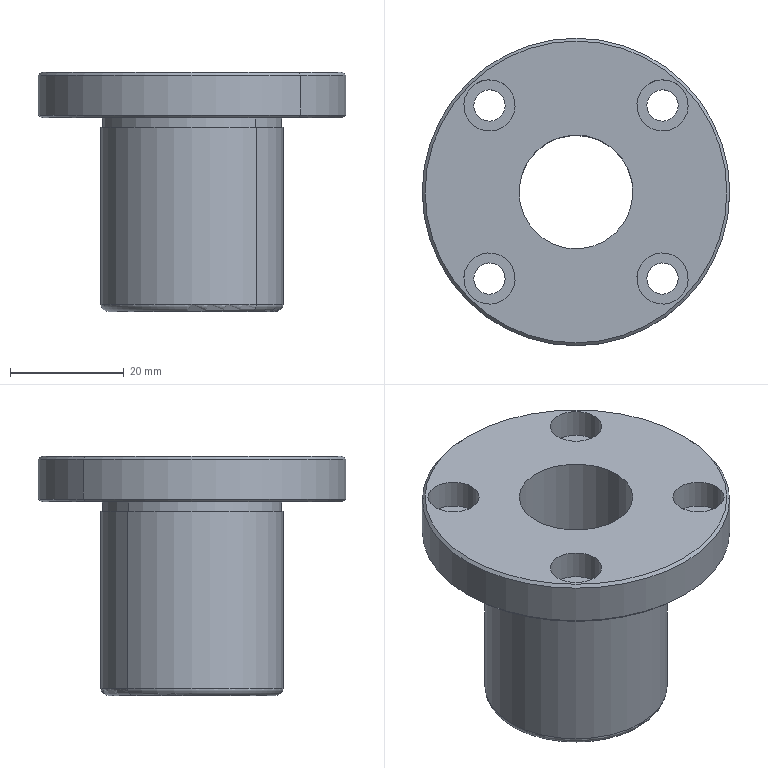Component | SolidWorks | SL010-RightStreamline-1-1_SL010-C-LHFR20-2-1-1 | 1 solid | 38 faces | box 54 x 54 x 42 mm | volume 30780 mm3 | cylinder 24 | plane 8 | cone 4 | torus 2 | commonest cylinder face diameters 9 x8 5.5 x8 54 x2 31.5 x2 32 x2 20 x2
STEP:
#1=COLOUR_RGB('',0.7922,0.8196,0.9333);
#2=FILL_AREA_STYLE_COLOUR('',#1);
#3=FILL_AREA_STYLE('',(#2));
#4=SURFACE_STYLE_FILL_AREA(#3);
#5=SURFACE_SIDE_STYLE('',(#4));
#6=SURFACE_STYLE_USAGE(.BOTH.,#5);
#7=PRESENTATION_STYLE_ASSIGNMENT((#6));
#8=CARTESIAN_POINT('',(27.442,-8.344,-12.328));
#9=VERTEX_POINT('',#8);
#10=CARTESIAN_POINT('',(27.692,-8.594,-12.328));
#11=VERTEX_POINT('',#10);
#12=CARTESIAN_POINT('',(27.567,-8.469,-12.328));
#13=DIRECTION('',(0.,0.,1.));
#14=DIRECTION('',(0.7071,-0.7071,0.));
#15=AXIS2_PLACEMENT_3D('',#12,#13,#14);
#16=CIRCLE('',#15,0.1772);
#17=EDGE_CURVE('',#9,#11,#16,.T.);
#18=ORIENTED_EDGE('',*,*,#17,.F.);
#19=CARTESIAN_POINT('',(27.442,-8.344,-12.127));
#20=VERTEX_POINT('',#19);
#21=CARTESIAN_POINT('',(27.442,-8.344,-12.127));
#22=DIRECTION('',(0.,0.,1.));
#23=VECTOR('',#22,39.37);
#24=LINE('',#21,#23);
#25=EDGE_CURVE('',#9,#20,#24,.T.);
#26=ORIENTED_EDGE('',*,*,#25,.T.);
#27=CARTESIAN_POINT('',(27.692,-8.594,-12.127));
#28=VERTEX_POINT('',#27);
#29=CARTESIAN_POINT('',(27.567,-8.469,-12.127));
#30=DIRECTION('',(0.,0.,1.));
#31=DIRECTION('',(0.7071,-0.7071,0.));
#32=AXIS2_PLACEMENT_3D('',#29,#30,#31);
#33=CIRCLE('',#32,0.1772);
#34=EDGE_CURVE('',#20,#28,#33,.T.);
#35=ORIENTED_EDGE('',*,*,#34,.T.);
#36=CARTESIAN_POINT('',(27.692,-8.594,-12.127));
#37=DIRECTION('',(0.,0.,1.));
#38=VECTOR('',#37,39.37);
#39=LINE('',#36,#38);
#40=EDGE_CURVE('',#11,#28,#39,.T.);
#41=ORIENTED_EDGE('',*,*,#40,.F.);
#42=EDGE_LOOP('',(#18,#26,#35,#41));
#43=FACE_OUTER_BOUND('',#42,.T.);
#44=CARTESIAN_POINT('',(27.567,-8.469,-12.127));
#45=DIRECTION('',(0.,0.,1.));
#46=DIRECTION('',(0.7071,-0.7071,0.));
#47=AXIS2_PLACEMENT_3D('',#44,#45,#46);
#48=CYLINDRICAL_SURFACE('',#47,0.1772);
#49=ADVANCED_FACE('',(#43),#48,.F.);
#50=CARTESIAN_POINT('',(27.49,-8.392,-12.442));
#51=VERTEX_POINT('',#50);
#52=CARTESIAN_POINT('',(27.644,-8.545,-12.442));
#53=VERTEX_POINT('',#52);
#54=CARTESIAN_POINT('',(27.567,-8.469,-12.442));
#55=DIRECTION('',(0.,0.,1.));
#56=DIRECTION('',(0.7071,-0.7071,0.));
#57=AXIS2_PLACEMENT_3D('',#54,#55,#56);
#58=CIRCLE('',#57,0.1083);
#59=EDGE_CURVE('',#51,#53,#58,.T.);
#60=ORIENTED_EDGE('',*,*,#59,.F.);
#61=CARTESIAN_POINT('',(27.49,-8.392,-12.328));
#62=VERTEX_POINT('',#61);
#63=CARTESIAN_POINT('',(27.49,-8.392,-12.127));
#64=DIRECTION('',(0.,0.,1.));
#65=VECTOR('',#64,39.37);
#66=LINE('',#63,#65);
#67=EDGE_CURVE('',#51,#62,#66,.T.);
#68=ORIENTED_EDGE('',*,*,#67,.T.);
#69=CARTESIAN_POINT('',(27.644,-8.545,-12.328));
#70=VERTEX_POINT('',#69);
#71=CARTESIAN_POINT('',(27.567,-8.469,-12.328));
#72=DIRECTION('',(0.,0.,1.));
#73=DIRECTION('',(0.7071,-0.7071,0.));
#74=AXIS2_PLACEMENT_3D('',#71,#72,#73);
#75=CIRCLE('',#74,0.1083);
#76=EDGE_CURVE('',#62,#70,#75,.T.);
#77=ORIENTED_EDGE('',*,*,#76,.T.);
#78=CARTESIAN_POINT('',(27.644,-8.545,-12.127));
#79=DIRECTION('',(0.,0.,1.));
#80=VECTOR('',#79,39.37);
#81=LINE('',#78,#80);
#82=EDGE_CURVE('',#53,#70,#81,.T.);
#83=ORIENTED_EDGE('',*,*,#82,.F.);
#84=EDGE_LOOP('',(#60,#68,#77,#83));
#85=FACE_OUTER_BOUND('',#84,.T.);
#86=CARTESIAN_POINT('',(27.567,-8.469,-12.127));
#87=DIRECTION('',(0.,0.,1.));
#88=DIRECTION('',(0.7071,-0.7071,0.));
#89=AXIS2_PLACEMENT_3D('',#86,#87,#88);
#90=CYLINDRICAL_SURFACE('',#89,0.1083);
#91=ADVANCED_FACE('',(#85),#90,.F.);
#92=CARTESIAN_POINT('',(26.245,-7.146,-12.328));
#93=VERTEX_POINT('',#92);
#94=CARTESIAN_POINT('',(26.495,-7.397,-12.328));
#95=VERTEX_POINT('',#94);
#96=CARTESIAN_POINT('',(26.37,-7.272,-12.328));
#97=DIRECTION('',(0.,0.,1.));
#98=DIRECTION('',(0.7071,-0.7071,0.));
#99=AXIS2_PLACEMENT_3D('',#96,#97,#98);
#100=CIRCLE('',#99,0.1772);
#101=EDGE_CURVE('',#93,#95,#100,.T.);
#102=ORIENTED_EDGE('',*,*,#101,.F.);
#103=CARTESIAN_POINT('',(26.245,-7.146,-12.127));
#104=VERTEX_POINT('',#103);
#105=CARTESIAN_POINT('',(26.245,-7.146,-12.127));
#106=DIRECTION('',(0.,0.,1.));
#107=VECTOR('',#106,39.37);
#108=LINE('',#105,#107);
#109=EDGE_CURVE('',#93,#104,#108,.T.);
#110=ORIENTED_EDGE('',*,*,#109,.T.);
#111=CARTESIAN_POINT('',(26.495,-7.397,-12.127));
#112=VERTEX_POINT('',#111);
#113=CARTESIAN_POINT('',(26.37,-7.272,-12.127));
#114=DIRECTION('',(0.,0.,1.));
#115=DIRECTION('',(0.7071,-0.7071,0.));
#116=AXIS2_PLACEMENT_3D('',#113,#114,#115);
#117=CIRCLE('',#116,0.1772);
#118=EDGE_CURVE('',#104,#112,#117,.T.);
#119=ORIENTED_EDGE('',*,*,#118,.T.);
#120=CARTESIAN_POINT('',(26.495,-7.397,-12.127));
#121=DIRECTION('',(0.,0.,1.));
#122=VECTOR('',#121,39.37);
#123=LINE('',#120,#122);
#124=EDGE_CURVE('',#95,#112,#123,.T.);
#125=ORIENTED_EDGE('',*,*,#124,.F.);
#126=EDGE_LOOP('',(#102,#110,#119,#125));
#127=FACE_OUTER_BOUND('',#126,.T.);
#128=CARTESIAN_POINT('',(26.37,-7.272,-12.127));
#129=DIRECTION('',(0.,0.,1.));
#130=DIRECTION('',(0.7071,-0.7071,0.));
#131=AXIS2_PLACEMENT_3D('',#128,#129,#130);
#132=CYLINDRICAL_SURFACE('',#131,0.1772);
#133=ADVANCED_FACE('',(#127),#132,.F.);
#134=CARTESIAN_POINT('',(26.293,-7.195,-12.442));
#135=VERTEX_POINT('',#134);
#136=CARTESIAN_POINT('',(26.447,-7.348,-12.442));
#137=VERTEX_POINT('',#136);
#138=CARTESIAN_POINT('',(26.37,-7.272,-12.442));
#139=DIRECTION('',(0.,0.,1.));
#140=DIRECTION('',(0.7071,-0.7071,0.));
#141=AXIS2_PLACEMENT_3D('',#138,#139,#140);
#142=CIRCLE('',#141,0.1083);
#143=EDGE_CURVE('',#135,#137,#142,.T.);
#144=ORIENTED_EDGE('',*,*,#143,.F.);
#145=CARTESIAN_POINT('',(26.293,-7.195,-12.328));
#146=VERTEX_POINT('',#145);
#147=CARTESIAN_POINT('',(26.293,-7.195,-12.127));
#148=DIRECTION('',(0.,0.,1.));
#149=VECTOR('',#148,39.37);
#150=LINE('',#147,#149);
#151=EDGE_CURVE('',#135,#146,#150,.T.);
#152=ORIENTED_EDGE('',*,*,#151,.T.);
#153=CARTESIAN_POINT('',(26.447,-7.348,-12.328));
#154=VERTEX_POINT('',#153);
#155=CARTESIAN_POINT('',(26.37,-7.272,-12.328));
#156=DIRECTION('',(0.,0.,1.));
#157=DIRECTION('',(0.7071,-0.7071,0.));
#158=AXIS2_PLACEMENT_3D('',#155,#156,#157);
#159=CIRCLE('',#158,0.1083);
#160=EDGE_CURVE('',#146,#154,#159,.T.);
#161=ORIENTED_EDGE('',*,*,#160,.T.);
#162=CARTESIAN_POINT('',(26.447,-7.348,-12.127));
#163=DIRECTION('',(0.,0.,1.));
#164=VECTOR('',#163,39.37);
#165=LINE('',#162,#164);
#166=EDGE_CURVE('',#137,#154,#165,.T.);
#167=ORIENTED_EDGE('',*,*,#166,.F.);
#168=EDGE_LOOP('',(#144,#152,#161,#167));
#169=FACE_OUTER_BOUND('',#168,.T.);
#170=CARTESIAN_POINT('',(26.37,-7.272,-12.127));
#171=DIRECTION('',(0.,0.,1.));
#172=DIRECTION('',(0.7071,-0.7071,0.));
#173=AXIS2_PLACEMENT_3D('',#170,#171,#172);
#174=CYLINDRICAL_SURFACE('',#173,0.1083);
#175=ADVANCED_FACE('',(#169),#174,.F.);
#176=CARTESIAN_POINT('',(26.245,-8.344,-12.328));
#177=VERTEX_POINT('',#176);
#178=CARTESIAN_POINT('',(26.495,-8.594,-12.328));
#179=VERTEX_POINT('',#178);
#180=CARTESIAN_POINT('',(26.37,-8.469,-12.328));
#181=DIRECTION('',(0.,0.,1.));
#182=DIRECTION('',(0.7071,-0.7071,0.));
#183=AXIS2_PLACEMENT_3D('',#180,#181,#182);
#184=CIRCLE('',#183,0.1772);
#185=EDGE_CURVE('',#177,#179,#184,.T.);
#186=ORIENTED_EDGE('',*,*,#185,.F.);
#187=CARTESIAN_POINT('',(26.245,-8.344,-12.127));
#188=VERTEX_POINT('',#187);
#189=CARTESIAN_POINT('',(26.245,-8.344,-12.127));
#190=DIRECTION('',(0.,0.,1.));
#191=VECTOR('',#190,39.37);
#192=LINE('',#189,#191);
#193=EDGE_CURVE('',#177,#188,#192,.T.);
#194=ORIENTED_EDGE('',*,*,#193,.T.);
#195=CARTESIAN_POINT('',(26.495,-8.594,-12.127));
#196=VERTEX_POINT('',#195);
#197=CARTESIAN_POINT('',(26.37,-8.469,-12.127));
#198=DIRECTION('',(0.,0.,1.));
#199=DIRECTION('',(0.7071,-0.7071,0.));
#200=AXIS2_PLACEMENT_3D('',#197,#198,#199);
#201=CIRCLE('',#200,0.1772);
#202=EDGE_CURVE('',#188,#196,#201,.T.);
#203=ORIENTED_EDGE('',*,*,#202,.T.);
#204=CARTESIAN_POINT('',(26.495,-8.594,-12.127));
#205=DIRECTION('',(0.,0.,1.));
#206=VECTOR('',#205,39.37);
#207=LINE('',#204,#206);
#208=EDGE_CURVE('',#179,#196,#207,.T.);
#209=ORIENTED_EDGE('',*,*,#208,.F.);
#210=EDGE_LOOP('',(#186,#194,#203,#209));
#211=FACE_OUTER_BOUND('',#210,.T.);
#212=CARTESIAN_POINT('',(26.37,-8.469,-12.127));
#213=DIRECTION('',(0.,0.,1.));
#214=DIRECTION('',(0.7071,-0.7071,0.));
#215=AXIS2_PLACEMENT_3D('',#212,#213,#214);
#216=CYLINDRICAL_SURFACE('',#215,0.1772);
#217=ADVANCED_FACE('',(#211),#216,.F.);
#218=CARTESIAN_POINT('',(26.293,-8.392,-12.442));
#219=VERTEX_POINT('',#218);
#220=CARTESIAN_POINT('',(26.447,-8.545,-12.442));
#221=VERTEX_POINT('',#220);
#222=CARTESIAN_POINT('',(26.37,-8.469,-12.442));
#223=DIRECTION('',(0.,0.,1.));
#224=DIRECTION('',(0.7071,-0.7071,0.));
#225=AXIS2_PLACEMENT_3D('',#222,#223,#224);
#226=CIRCLE('',#225,0.1083);
#227=EDGE_CURVE('',#219,#221,#226,.T.);
#228=ORIENTED_EDGE('',*,*,#227,.F.);
#229=CARTESIAN_POINT('',(26.293,-8.392,-12.328));
#230=VERTEX_POINT('',#229);
#231=CARTESIAN_POINT('',(26.293,-8.392,-12.127));
#232=DIRECTION('',(0.,0.,1.));
#233=VECTOR('',#232,39.37);
#234=LINE('',#231,#233);
#235=EDGE_CURVE('',#219,#230,#234,.T.);
#236=ORIENTED_EDGE('',*,*,#235,.T.);
#237=CARTESIAN_POINT('',(26.447,-8.545,-12.328));
#238=VERTEX_POINT('',#237);
#239=CARTESIAN_POINT('',(26.37,-8.469,-12.328));
#240=DIRECTION('',(0.,0.,1.));
#241=DIRECTION('',(0.7071,-0.7071,0.));
#242=AXIS2_PLACEMENT_3D('',#239,#240,#241);
#243=CIRCLE('',#242,0.1083);
#244=EDGE_CURVE('',#230,#238,#243,.T.);
#245=ORIENTED_EDGE('',*,*,#244,.T.);
#246=CARTESIAN_POINT('',(26.447,-8.545,-12.127));
#247=DIRECTION('',(0.,0.,1.));
#248=VECTOR('',#247,39.37);
#249=LINE('',#246,#248);
#250=EDGE_CURVE('',#221,#238,#249,.T.);
#251=ORIENTED_EDGE('',*,*,#250,.F.);
#252=EDGE_LOOP('',(#228,#236,#245,#251));
#253=FACE_OUTER_BOUND('',#252,.T.);
#254=CARTESIAN_POINT('',(26.37,-8.469,-12.127));
#255=DIRECTION('',(0.,0.,1.));
#256=DIRECTION('',(0.7071,-0.7071,0.));
#257=AXIS2_PLACEMENT_3D('',#254,#255,#256);
#258=CYLINDRICAL_SURFACE('',#257,0.1083);
#259=ADVANCED_FACE('',(#253),#258,.F.);
#260=CARTESIAN_POINT('',(27.442,-7.146,-12.328));
#261=VERTEX_POINT('',#260);
#262=CARTESIAN_POINT('',(27.692,-7.397,-12.328));
#263=VERTEX_POINT('',#262);
#264=CARTESIAN_POINT('',(27.567,-7.272,-12.328));
#265=DIRECTION('',(0.,0.,1.));
#266=DIRECTION('',(0.7071,-0.7071,0.));
#267=AXIS2_PLACEMENT_3D('',#264,#265,#266);
#268=CIRCLE('',#267,0.1772);
#269=EDGE_CURVE('',#261,#263,#268,.T.);
#270=ORIENTED_EDGE('',*,*,#269,.F.);
#271=CARTESIAN_POINT('',(27.442,-7.146,-12.127));
#272=VERTEX_POINT('',#271);
#273=CARTESIAN_POINT('',(27.442,-7.146,-12.127));
#274=DIRECTION('',(0.,0.,1.));
#275=VECTOR('',#274,39.37);
#276=LINE('',#273,#275);
#277=EDGE_CURVE('',#261,#272,#276,.T.);
#278=ORIENTED_EDGE('',*,*,#277,.T.);
#279=CARTESIAN_POINT('',(27.692,-7.397,-12.127));
#280=VERTEX_POINT('',#279);
#281=CARTESIAN_POINT('',(27.567,-7.272,-12.127));
#282=DIRECTION('',(0.,0.,1.));
#283=DIRECTION('',(0.7071,-0.7071,0.));
#284=AXIS2_PLACEMENT_3D('',#281,#282,#283);
#285=CIRCLE('',#284,0.1772);
#286=EDGE_CURVE('',#272,#280,#285,.T.);
#287=ORIENTED_EDGE('',*,*,#286,.T.);
#288=CARTESIAN_POINT('',(27.692,-7.397,-12.127));
#289=DIRECTION('',(0.,0.,1.));
#290=VECTOR('',#289,39.37);
#291=LINE('',#288,#290);
#292=EDGE_CURVE('',#263,#280,#291,.T.);
#293=ORIENTED_EDGE('',*,*,#292,.F.);
#294=EDGE_LOOP('',(#270,#278,#287,#293));
#295=FACE_OUTER_BOUND('',#294,.T.);
#296=CARTESIAN_POINT('',(27.567,-7.272,-12.127));
#297=DIRECTION('',(0.,0.,1.));
#298=DIRECTION('',(0.7071,-0.7071,0.));
#299=AXIS2_PLACEMENT_3D('',#296,#297,#298);
#300=CYLINDRICAL_SURFACE('',#299,0.1772);
#301=ADVANCED_FACE('',(#295),#300,.F.);
#302=CARTESIAN_POINT('',(27.49,-7.195,-12.442));
#303=VERTEX_POINT('',#302);
#304=CARTESIAN_POINT('',(27.644,-7.348,-12.442));
#305=VERTEX_POINT('',#304);
#306=CARTESIAN_POINT('',(27.567,-7.272,-12.442));
#307=DIRECTION('',(0.,0.,1.));
#308=DIRECTION('',(0.7071,-0.7071,0.));
#309=AXIS2_PLACEMENT_3D('',#306,#307,#308);
#310=CIRCLE('',#309,0.1083);
#311=EDGE_CURVE('',#303,#305,#310,.T.);
#312=ORIENTED_EDGE('',*,*,#311,.F.);
#313=CARTESIAN_POINT('',(27.49,-7.195,-12.328));
#314=VERTEX_POINT('',#313);
#315=CARTESIAN_POINT('',(27.49,-7.195,-12.127));
#316=DIRECTION('',(0.,0.,1.));
#317=VECTOR('',#316,39.37);
#318=LINE('',#315,#317);
#319=EDGE_CURVE('',#303,#314,#318,.T.);
#320=ORIENTED_EDGE('',*,*,#319,.T.);
#321=CARTESIAN_POINT('',(27.644,-7.348,-12.328));
#322=VERTEX_POINT('',#321);
#323=CARTESIAN_POINT('',(27.567,-7.272,-12.328));
#324=DIRECTION('',(0.,0.,1.));
#325=DIRECTION('',(0.7071,-0.7071,0.));
#326=AXIS2_PLACEMENT_3D('',#323,#324,#325);
#327=CIRCLE('',#326,0.1083);
#328=EDGE_CURVE('',#314,#322,#327,.T.);
#329=ORIENTED_EDGE('',*,*,#328,.T.);
#330=CARTESIAN_POINT('',(27.644,-7.348,-12.127));
#331=DIRECTION('',(0.,0.,1.));
#332=VECTOR('',#331,39.37);
#333=LINE('',#330,#332);
#334=EDGE_CURVE('',#305,#322,#333,.T.);
#335=ORIENTED_EDGE('',*,*,#334,.F.);
#336=EDGE_LOOP('',(#312,#320,#329,#335));
#337=FACE_OUTER_BOUND('',#336,.T.);
#338=CARTESIAN_POINT('',(27.567,-7.272,-12.127));
#339=DIRECTION('',(0.,0.,1.));
#340=DIRECTION('',(0.7071,-0.7071,0.));
#341=AXIS2_PLACEMENT_3D('',#338,#339,#340);
#342=CYLINDRICAL_SURFACE('',#341,0.1083);
#343=ADVANCED_FACE('',(#337),#342,.F.);
#344=CARTESIAN_POINT('',(27.72,-8.622,-12.423));
#345=VERTEX_POINT('',#344);
#346=CARTESIAN_POINT('',(26.217,-7.119,-12.423));
#347=VERTEX_POINT('',#346);
#348=CARTESIAN_POINT('',(26.969,-7.87,-12.423));
#349=DIRECTION('',(0.,0.,1.));
#350=DIRECTION('',(0.7071,-0.7071,0.));
#351=AXIS2_PLACEMENT_3D('',#348,#349,#350);
#352=CIRCLE('',#351,1.063);
#353=EDGE_CURVE('',#345,#347,#352,.T.);
#354=ORIENTED_EDGE('',*,*,#353,.T.);
#355=CARTESIAN_POINT('',(26.217,-7.119,-12.147));
#356=VERTEX_POINT('',#355);
#357=CARTESIAN_POINT('',(26.217,-7.119,-13.781));
#358=DIRECTION('',(0.,0.,1.));
#359=VECTOR('',#358,39.37);
#360=LINE('',#357,#359);
#361=EDGE_CURVE('',#347,#356,#360,.T.);
#362=ORIENTED_EDGE('',*,*,#361,.T.);
#363=CARTESIAN_POINT('',(27.72,-8.622,-12.147));
#364=VERTEX_POINT('',#363);
#365=CARTESIAN_POINT('',(26.969,-7.87,-12.147));
#366=DIRECTION('',(0.,0.,1.));
#367=DIRECTION('',(0.7071,-0.7071,0.));
#368=AXIS2_PLACEMENT_3D('',#365,#366,#367);
#369=CIRCLE('',#368,1.063);
#370=EDGE_CURVE('',#364,#356,#369,.T.);
#371=ORIENTED_EDGE('',*,*,#370,.F.);
#372=CARTESIAN_POINT('',(27.72,-8.622,-13.781));
#373=DIRECTION('',(0.,0.,1.));
#374=VECTOR('',#373,39.37);
#375=LINE('',#372,#374);
#376=EDGE_CURVE('',#345,#364,#375,.T.);
#377=ORIENTED_EDGE('',*,*,#376,.F.);
#378=EDGE_LOOP('',(#354,#362,#371,#377));
#379=FACE_OUTER_BOUND('',#378,.T.);
#380=CARTESIAN_POINT('',(26.969,-7.87,-13.781));
#381=DIRECTION('',(0.,0.,1.));
#382=DIRECTION('',(0.7071,-0.7071,0.));
#383=AXIS2_PLACEMENT_3D('',#380,#381,#382);
#384=CYLINDRICAL_SURFACE('',#383,1.063);
#385=ADVANCED_FACE('',(#379),#384,.T.);
#386=CARTESIAN_POINT('',(27.706,-8.608,-12.442));
#387=VERTEX_POINT('',#386);
#388=CARTESIAN_POINT('',(26.231,-7.133,-12.442));
#389=VERTEX_POINT('',#388);
#390=CARTESIAN_POINT('',(26.969,-7.87,-12.442));
#391=DIRECTION('',(0.,0.,1.));
#392=DIRECTION('',(0.7071,-0.7071,0.));
#393=AXIS2_PLACEMENT_3D('',#390,#391,#392);
#394=CIRCLE('',#393,1.043);
#395=EDGE_CURVE('',#387,#389,#394,.T.);
#396=ORIENTED_EDGE('',*,*,#395,.T.);
#397=CARTESIAN_POINT('',(26.231,-7.133,-12.442));
#398=DIRECTION('',(-0.5,0.5,0.7071));
#399=VECTOR('',#398,39.37);
#400=LINE('',#397,#399);
#401=EDGE_CURVE('',#389,#347,#400,.T.);
#402=ORIENTED_EDGE('',*,*,#401,.T.);
#403=ORIENTED_EDGE('',*,*,#353,.F.);
#404=CARTESIAN_POINT('',(27.706,-8.608,-12.442));
#405=DIRECTION('',(0.5,-0.5,0.7071));
#406=VECTOR('',#405,39.37);
#407=LINE('',#404,#406);
#408=EDGE_CURVE('',#387,#345,#407,.T.);
#409=ORIENTED_EDGE('',*,*,#408,.F.);
#410=EDGE_LOOP('',(#396,#402,#403,#409));
#411=FACE_OUTER_BOUND('',#410,.T.);
#412=CARTESIAN_POINT('',(26.969,-7.87,-12.442));
#413=DIRECTION('',(0.,0.,1.));
#414=DIRECTION('',(0.7071,-0.7071,0.));
#415=AXIS2_PLACEMENT_3D('',#412,#413,#414);
#416=CONICAL_SURFACE('',#415,1.043,0.7854);
#417=ADVANCED_FACE('',(#411),#416,.T.);
#418=CARTESIAN_POINT('',(27.407,-8.309,-12.505));
#419=VERTEX_POINT('',#418);
#420=CARTESIAN_POINT('',(26.53,-7.432,-12.505));
#421=VERTEX_POINT('',#420);
#422=CARTESIAN_POINT('',(26.969,-7.87,-12.505));
#423=DIRECTION('',(0.,0.,1.));
#424=DIRECTION('',(0.7071,-0.7071,0.));
#425=AXIS2_PLACEMENT_3D('',#422,#423,#424);
#426=CIRCLE('',#425,0.6201);
#427=EDGE_CURVE('',#419,#421,#426,.T.);
#428=ORIENTED_EDGE('',*,*,#427,.T.);
#429=CARTESIAN_POINT('',(26.53,-7.432,-12.442));
#430=VERTEX_POINT('',#429);
#431=CARTESIAN_POINT('',(26.53,-7.432,-13.781));
#432=DIRECTION('',(0.,0.,1.));
#433=VECTOR('',#432,39.37);
#434=LINE('',#431,#433);
#435=EDGE_CURVE('',#421,#430,#434,.T.);
#436=ORIENTED_EDGE('',*,*,#435,.T.);
#437=CARTESIAN_POINT('',(27.407,-8.309,-12.442));
#438=VERTEX_POINT('',#437);
#439=CARTESIAN_POINT('',(26.969,-7.87,-12.442));
#440=DIRECTION('',(0.,0.,1.));
#441=DIRECTION('',(0.7071,-0.7071,0.));
#442=AXIS2_PLACEMENT_3D('',#439,#440,#441);
#443=CIRCLE('',#442,0.6201);
#444=EDGE_CURVE('',#438,#430,#443,.T.);
#445=ORIENTED_EDGE('',*,*,#444,.F.);
#446=CARTESIAN_POINT('',(27.407,-8.309,-13.781));
#447=DIRECTION('',(0.,0.,1.));
#448=VECTOR('',#447,39.37);
#449=LINE('',#446,#448);
#450=EDGE_CURVE('',#419,#438,#449,.T.);
#451=ORIENTED_EDGE('',*,*,#450,.F.);
#452=EDGE_LOOP('',(#428,#436,#445,#451));
#453=FACE_OUTER_BOUND('',#452,.T.);
#454=CARTESIAN_POINT('',(26.969,-7.87,-13.781));
#455=DIRECTION('',(0.,0.,1.));
#456=DIRECTION('',(0.7071,-0.7071,0.));
#457=AXIS2_PLACEMENT_3D('',#454,#455,#456);
#458=CYLINDRICAL_SURFACE('',#457,0.6201);
#459=ADVANCED_FACE('',(#453),#458,.T.);
#460=CARTESIAN_POINT('',(27.414,-8.316,-13.73));
#461=VERTEX_POINT('',#460);
#462=CARTESIAN_POINT('',(26.523,-7.425,-13.73));
#463=VERTEX_POINT('',#462);
#464=CARTESIAN_POINT('',(26.969,-7.87,-13.73));
#465=DIRECTION('',(0.,0.,1.));
#466=DIRECTION('',(0.7071,-0.7071,0.));
#467=AXIS2_PLACEMENT_3D('',#464,#465,#466);
#468=CIRCLE('',#467,0.6299);
#469=EDGE_CURVE('',#461,#463,#468,.T.);
#470=ORIENTED_EDGE('',*,*,#469,.T.);
#471=CARTESIAN_POINT('',(26.523,-7.425,-12.505));
#472=VERTEX_POINT('',#471);
#473=CARTESIAN_POINT('',(26.523,-7.425,-13.781));
#474=DIRECTION('',(0.,0.,1.));
#475=VECTOR('',#474,39.37);
#476=LINE('',#473,#475);
#477=EDGE_CURVE('',#463,#472,#476,.T.);
#478=ORIENTED_EDGE('',*,*,#477,.T.);
#479=CARTESIAN_POINT('',(27.414,-8.316,-12.505));
#480=VERTEX_POINT('',#479);
#481=CARTESIAN_POINT('',(26.969,-7.87,-12.505));
#482=DIRECTION('',(0.,0.,1.));
#483=DIRECTION('',(0.7071,-0.7071,0.));
#484=AXIS2_PLACEMENT_3D('',#481,#482,#483);
#485=CIRCLE('',#484,0.6299);
#486=EDGE_CURVE('',#480,#472,#485,.T.);
#487=ORIENTED_EDGE('',*,*,#486,.F.);
#488=CARTESIAN_POINT('',(27.414,-8.316,-13.781));
#489=DIRECTION('',(0.,0.,1.));
#490=VECTOR('',#489,39.37);
#491=LINE('',#488,#490);
#492=EDGE_CURVE('',#461,#480,#491,.T.);
#493=ORIENTED_EDGE('',*,*,#492,.F.);
#494=EDGE_LOOP('',(#470,#478,#487,#493));
#495=FACE_OUTER_BOUND('',#494,.T.);
#496=CARTESIAN_POINT('',(26.969,-7.87,-13.781));
#497=DIRECTION('',(0.,0.,1.));
#498=DIRECTION('',(0.7071,-0.7071,0.));
#499=AXIS2_PLACEMENT_3D('',#496,#497,#498);
#500=CYLINDRICAL_SURFACE('',#499,0.6299);
#501=ADVANCED_FACE('',(#495),#500,.T.);
#502=CARTESIAN_POINT('',(27.378,-8.279,-13.781));
#503=VERTEX_POINT('',#502);
#504=CARTESIAN_POINT('',(26.559,-7.461,-13.781));
#505=VERTEX_POINT('',#504);
#506=CARTESIAN_POINT('',(26.969,-7.87,-13.781));
#507=DIRECTION('',(0.,0.,1.));
#508=DIRECTION('',(0.7071,-0.7071,0.));
#509=AXIS2_PLACEMENT_3D('',#506,#507,#508);
#510=CIRCLE('',#509,0.5787);
#511=EDGE_CURVE('',#503,#505,#510,.T.);
#512=ORIENTED_EDGE('',*,*,#511,.T.);
#513=CARTESIAN_POINT('',(26.559,-7.461,-13.73));
#514=DIRECTION('',(0.7071,0.7071,-0.));
#515=DIRECTION('',(-0.7071,0.7071,0.));
#516=AXIS2_PLACEMENT_3D('',#513,#514,#515);
#517=CIRCLE('',#516,0.05118);
#518=EDGE_CURVE('',#505,#463,#517,.T.);
#519=ORIENTED_EDGE('',*,*,#518,.T.);
#520=ORIENTED_EDGE('',*,*,#469,.F.);
#521=CARTESIAN_POINT('',(27.378,-8.279,-13.73));
#522=DIRECTION('',(-0.7071,-0.7071,0.));
#523=DIRECTION('',(0.7071,-0.7071,0.));
#524=AXIS2_PLACEMENT_3D('',#521,#522,#523);
#525=CIRCLE('',#524,0.05118);
#526=EDGE_CURVE('',#503,#461,#525,.T.);
#527=ORIENTED_EDGE('',*,*,#526,.F.);
#528=EDGE_LOOP('',(#512,#519,#520,#527));
#529=FACE_OUTER_BOUND('',#528,.T.);
#530=CARTESIAN_POINT('',(26.969,-7.87,-13.73));
#531=DIRECTION('',(0.,0.,1.));
#532=DIRECTION('',(0.7071,-0.7071,0.));
#533=AXIS2_PLACEMENT_3D('',#530,#531,#532);
#534=TOROIDAL_SURFACE('',#533,0.5787,0.05118);
#535=ADVANCED_FACE('',(#529),#534,.T.);
#536=CARTESIAN_POINT('',(26.69,-7.592,-13.781));
#537=VERTEX_POINT('',#536);
#538=CARTESIAN_POINT('',(27.247,-8.149,-13.781));
#539=VERTEX_POINT('',#538);
#540=CARTESIAN_POINT('',(26.969,-7.87,-13.781));
#541=DIRECTION('',(0.,0.,1.));
#542=DIRECTION('',(0.7071,-0.7071,0.));
#543=AXIS2_PLACEMENT_3D('',#540,#541,#542);
#544=CIRCLE('',#543,0.3937);
#545=EDGE_CURVE('',#537,#539,#544,.T.);
#546=ORIENTED_EDGE('',*,*,#545,.F.);
#547=CARTESIAN_POINT('',(26.69,-7.592,-12.127));
#548=VERTEX_POINT('',#547);
#549=CARTESIAN_POINT('',(26.69,-7.592,-13.781));
#550=DIRECTION('',(0.,0.,1.));
#551=VECTOR('',#550,39.37);
#552=LINE('',#549,#551);
#553=EDGE_CURVE('',#537,#548,#552,.T.);
#554=ORIENTED_EDGE('',*,*,#553,.T.);
#555=CARTESIAN_POINT('',(27.247,-8.149,-12.127));
#556=VERTEX_POINT('',#555);
#557=CARTESIAN_POINT('',(26.969,-7.87,-12.127));
#558=DIRECTION('',(0.,0.,1.));
#559=DIRECTION('',(0.7071,-0.7071,0.));
#560=AXIS2_PLACEMENT_3D('',#557,#558,#559);
#561=CIRCLE('',#560,0.3937);
#562=EDGE_CURVE('',#548,#556,#561,.T.);
#563=ORIENTED_EDGE('',*,*,#562,.T.);
#564=CARTESIAN_POINT('',(27.247,-8.149,-13.781));
#565=DIRECTION('',(0.,0.,1.));
#566=VECTOR('',#565,39.37);
#567=LINE('',#564,#566);
#568=EDGE_CURVE('',#539,#556,#567,.T.);
#569=ORIENTED_EDGE('',*,*,#568,.F.);
#570=EDGE_LOOP('',(#546,#554,#563,#569));
#571=FACE_OUTER_BOUND('',#570,.T.);
#572=CARTESIAN_POINT('',(26.969,-7.87,-13.781));
#573=DIRECTION('',(0.,0.,1.));
#574=DIRECTION('',(0.7071,-0.7071,0.));
#575=AXIS2_PLACEMENT_3D('',#572,#573,#574);
#576=CYLINDRICAL_SURFACE('',#575,0.3937);
#577=ADVANCED_FACE('',(#571),#576,.F.);
#578=CARTESIAN_POINT('',(27.706,-8.608,-12.127));
#579=VERTEX_POINT('',#578);
#580=CARTESIAN_POINT('',(26.231,-7.133,-12.127));
#581=VERTEX_POINT('',#580);
#582=CARTESIAN_POINT('',(26.969,-7.87,-12.127));
#583=DIRECTION('',(0.,0.,1.));
#584=DIRECTION('',(0.7071,-0.7071,0.));
#585=AXIS2_PLACEMENT_3D('',#582,#583,#584);
#586=CIRCLE('',#585,1.043);
#587=EDGE_CURVE('',#579,#581,#586,.T.);
#588=ORIENTED_EDGE('',*,*,#587,.F.);
#589=CARTESIAN_POINT('',(27.72,-8.622,-12.147));
#590=DIRECTION('',(0.5,-0.5,-0.7071));
#591=VECTOR('',#590,39.37);
#592=LINE('',#589,#591);
#593=EDGE_CURVE('',#579,#364,#592,.T.);
#594=ORIENTED_EDGE('',*,*,#593,.T.);
#595=ORIENTED_EDGE('',*,*,#370,.T.);
#596=CARTESIAN_POINT('',(26.217,-7.119,-12.147));
#597=DIRECTION('',(-0.5,0.5,-0.7071));
#598=VECTOR('',#597,39.37);
#599=LINE('',#596,#598);
#600=EDGE_CURVE('',#581,#356,#599,.T.);
#601=ORIENTED_EDGE('',*,*,#600,.F.);
#602=EDGE_LOOP('',(#588,#594,#595,#601));
#603=FACE_OUTER_BOUND('',#602,.T.);
#604=CARTESIAN_POINT('',(26.969,-7.87,-12.147));
#605=DIRECTION('',(-0.,-0.,-1.));
#606=DIRECTION('',(-0.7071,0.7071,0.));
#607=AXIS2_PLACEMENT_3D('',#604,#605,#606);
#608=CONICAL_SURFACE('',#607,1.063,0.7854);
#609=ADVANCED_FACE('',(#603),#608,.T.);
#610=ORIENTED_EDGE('',*,*,#593,.F.);
#611=CARTESIAN_POINT('',(26.969,-7.87,-12.127));
#612=DIRECTION('',(0.,0.,1.));
#613=DIRECTION('',(0.7071,-0.7071,0.));
#614=AXIS2_PLACEMENT_3D('',#611,#612,#613);
#615=CIRCLE('',#614,1.043);
#616=EDGE_CURVE('',#581,#579,#615,.T.);
#617=ORIENTED_EDGE('',*,*,#616,.F.);
#618=ORIENTED_EDGE('',*,*,#600,.T.);
#619=CARTESIAN_POINT('',(26.969,-7.87,-12.147));
#620=DIRECTION('',(0.,0.,1.));
#621=DIRECTION('',(0.7071,-0.7071,0.));
#622=AXIS2_PLACEMENT_3D('',#619,#620,#621);
#623=CIRCLE('',#622,1.063);
#624=EDGE_CURVE('',#356,#364,#623,.T.);
#625=ORIENTED_EDGE('',*,*,#624,.T.);
#626=EDGE_LOOP('',(#610,#617,#618,#625));
#627=FACE_OUTER_BOUND('',#626,.T.);
#628=CARTESIAN_POINT('',(26.969,-7.87,-12.147));
#629=DIRECTION('',(-0.,-0.,-1.));
#630=DIRECTION('',(-0.7071,0.7071,0.));
#631=AXIS2_PLACEMENT_3D('',#628,#629,#630);
#632=CONICAL_SURFACE('',#631,1.063,0.7854);
#633=ADVANCED_FACE('',(#627),#632,.T.);
#634=CARTESIAN_POINT('',(27.567,-8.469,-12.127));
#635=DIRECTION('',(0.,0.,1.));
#636=DIRECTION('',(0.7071,-0.7071,0.));
#637=AXIS2_PLACEMENT_3D('',#634,#635,#636);
#638=CIRCLE('',#637,0.1772);
#639=EDGE_CURVE('',#28,#20,#638,.T.);
#640=ORIENTED_EDGE('',*,*,#639,.F.);
#641=ORIENTED_EDGE('',*,*,#34,.F.);
#642=EDGE_LOOP('',(#640,#641));
#643=FACE_BOUND('',#642,.T.);
#644=CARTESIAN_POINT('',(26.37,-7.272,-12.127));
#645=DIRECTION('',(0.,0.,1.));
#646=DIRECTION('',(0.7071,-0.7071,0.));
#647=AXIS2_PLACEMENT_3D('',#644,#645,#646);
#648=CIRCLE('',#647,0.1772);
#649=EDGE_CURVE('',#112,#104,#648,.T.);
#650=ORIENTED_EDGE('',*,*,#649,.F.);
#651=ORIENTED_EDGE('',*,*,#118,.F.);
#652=EDGE_LOOP('',(#650,#651));
#653=FACE_BOUND('',#652,.T.);
#654=CARTESIAN_POINT('',(26.37,-8.469,-12.127));
#655=DIRECTION('',(0.,0.,1.));
#656=DIRECTION('',(0.7071,-0.7071,0.));
#657=AXIS2_PLACEMENT_3D('',#654,#655,#656);
#658=CIRCLE('',#657,0.1772);
#659=EDGE_CURVE('',#196,#188,#658,.T.);
#660=ORIENTED_EDGE('',*,*,#659,.F.);
#661=ORIENTED_EDGE('',*,*,#202,.F.);
#662=EDGE_LOOP('',(#660,#661));
#663=FACE_BOUND('',#662,.T.);
#664=CARTESIAN_POINT('',(27.567,-7.272,-12.127));
#665=DIRECTION('',(0.,0.,1.));
#666=DIRECTION('',(0.7071,-0.7071,0.));
#667=AXIS2_PLACEMENT_3D('',#664,#665,#666);
#668=CIRCLE('',#667,0.1772);
#669=EDGE_CURVE('',#280,#272,#668,.T.);
#670=ORIENTED_EDGE('',*,*,#669,.F.);
#671=ORIENTED_EDGE('',*,*,#286,.F.);
#672=EDGE_LOOP('',(#670,#671));
#673=FACE_BOUND('',#672,.T.);
#674=CARTESIAN_POINT('',(26.969,-7.87,-12.127));
#675=DIRECTION('',(0.,0.,1.));
#676=DIRECTION('',(0.7071,-0.7071,0.));
#677=AXIS2_PLACEMENT_3D('',#674,#675,#676);
#678=CIRCLE('',#677,0.3937);
#679=EDGE_CURVE('',#556,#548,#678,.T.);
#680=ORIENTED_EDGE('',*,*,#679,.F.);
#681=ORIENTED_EDGE('',*,*,#562,.F.);
#682=EDGE_LOOP('',(#680,#681));
#683=FACE_BOUND('',#682,.T.);
#684=ORIENTED_EDGE('',*,*,#616,.T.);
#685=ORIENTED_EDGE('',*,*,#587,.T.);
#686=EDGE_LOOP('',(#684,#685));
#687=FACE_OUTER_BOUND('',#686,.T.);
#688=CARTESIAN_POINT('',(27.706,-7.133,-12.127));
#689=DIRECTION('',(-0.,-0.,-1.));
#690=DIRECTION('',(-0.7071,0.7071,-0.));
#691=AXIS2_PLACEMENT_3D('',#688,#689,#690);
#692=PLANE('',#691);
#693=ADVANCED_FACE('',(#643,#653,#663,#673,#683,#687),#692,.F.);
#694=ORIENTED_EDGE('',*,*,#553,.F.);
#695=CARTESIAN_POINT('',(26.969,-7.87,-13.781));
#696=DIRECTION('',(0.,0.,1.));
#697=DIRECTION('',(0.7071,-0.7071,0.));
#698=AXIS2_PLACEMENT_3D('',#695,#696,#697);
#699=CIRCLE('',#698,0.3937);
#700=EDGE_CURVE('',#539,#537,#699,.T.);
#701=ORIENTED_EDGE('',*,*,#700,.F.);
#702=ORIENTED_EDGE('',*,*,#568,.T.);
#703=ORIENTED_EDGE('',*,*,#679,.T.);
#704=EDGE_LOOP('',(#694,#701,#702,#703));
#705=FACE_OUTER_BOUND('',#704,.T.);
#706=CARTESIAN_POINT('',(26.969,-7.87,-13.781));
#707=DIRECTION('',(0.,0.,1.));
#708=DIRECTION('',(0.7071,-0.7071,0.));
#709=AXIS2_PLACEMENT_3D('',#706,#707,#708);
#710=CYLINDRICAL_SURFACE('',#709,0.3937);
#711=ADVANCED_FACE('',(#705),#710,.F.);
#712=ORIENTED_EDGE('',*,*,#511,.F.);
#713=CARTESIAN_POINT('',(26.969,-7.87,-13.781));
#714=DIRECTION('',(0.,0.,1.));
#715=DIRECTION('',(0.7071,-0.7071,0.));
#716=AXIS2_PLACEMENT_3D('',#713,#714,#715);
#717=CIRCLE('',#716,0.5787);
#718=EDGE_CURVE('',#505,#503,#717,.T.);
#719=ORIENTED_EDGE('',*,*,#718,.F.);
#720=EDGE_LOOP('',(#712,#719));
#721=FACE_OUTER_BOUND('',#720,.T.);
#722=ORIENTED_EDGE('',*,*,#700,.T.);
#723=ORIENTED_EDGE('',*,*,#545,.T.);
#724=EDGE_LOOP('',(#722,#723));
#725=FACE_BOUND('',#724,.T.);
#726=CARTESIAN_POINT('',(27.247,-7.592,-13.781));
#727=DIRECTION('',(0.,0.,1.));
#728=DIRECTION('',(0.7071,-0.7071,0.));
#729=AXIS2_PLACEMENT_3D('',#726,#727,#728);
#730=PLANE('',#729);
#731=ADVANCED_FACE('',(#721,#725),#730,.F.);
#732=ORIENTED_EDGE('',*,*,#518,.F.);
#733=ORIENTED_EDGE('',*,*,#718,.T.);
#734=ORIENTED_EDGE('',*,*,#526,.T.);
#735=CARTESIAN_POINT('',(26.969,-7.87,-13.73));
#736=DIRECTION('',(0.,0.,1.));
#737=DIRECTION('',(0.7071,-0.7071,0.));
#738=AXIS2_PLACEMENT_3D('',#735,#736,#737);
#739=CIRCLE('',#738,0.6299);
#740=EDGE_CURVE('',#463,#461,#739,.T.);
#741=ORIENTED_EDGE('',*,*,#740,.F.);
#742=EDGE_LOOP('',(#732,#733,#734,#741));
#743=FACE_OUTER_BOUND('',#742,.T.);
#744=CARTESIAN_POINT('',(26.969,-7.87,-13.73));
#745=DIRECTION('',(0.,0.,1.));
#746=DIRECTION('',(0.7071,-0.7071,0.));
#747=AXIS2_PLACEMENT_3D('',#744,#745,#746);
#748=TOROIDAL_SURFACE('',#747,0.5787,0.05118);
#749=ADVANCED_FACE('',(#743),#748,.T.);
#750=ORIENTED_EDGE('',*,*,#477,.F.);
#751=ORIENTED_EDGE('',*,*,#740,.T.);
#752=ORIENTED_EDGE('',*,*,#492,.T.);
#753=CARTESIAN_POINT('',(26.969,-7.87,-12.505));
#754=DIRECTION('',(0.,0.,1.));
#755=DIRECTION('',(0.7071,-0.7071,0.));
#756=AXIS2_PLACEMENT_3D('',#753,#754,#755);
#757=CIRCLE('',#756,0.6299);
#758=EDGE_CURVE('',#472,#480,#757,.T.);
#759=ORIENTED_EDGE('',*,*,#758,.F.);
#760=EDGE_LOOP('',(#750,#751,#752,#759));
#761=FACE_OUTER_BOUND('',#760,.T.);
#762=CARTESIAN_POINT('',(26.969,-7.87,-13.781));
#763=DIRECTION('',(0.,0.,1.));
#764=DIRECTION('',(0.7071,-0.7071,0.));
#765=AXIS2_PLACEMENT_3D('',#762,#763,#764);
#766=CYLINDRICAL_SURFACE('',#765,0.6299);
#767=ADVANCED_FACE('',(#761),#766,.T.);
#768=ORIENTED_EDGE('',*,*,#427,.F.);
#769=CARTESIAN_POINT('',(26.969,-7.87,-12.505));
#770=DIRECTION('',(0.,0.,1.));
#771=DIRECTION('',(0.7071,-0.7071,0.));
#772=AXIS2_PLACEMENT_3D('',#769,#770,#771);
#773=CIRCLE('',#772,0.6201);
#774=EDGE_CURVE('',#421,#419,#773,.T.);
#775=ORIENTED_EDGE('',*,*,#774,.F.);
#776=EDGE_LOOP('',(#768,#775));
#777=FACE_BOUND('',#776,.T.);
#778=ORIENTED_EDGE('',*,*,#486,.T.);
#779=ORIENTED_EDGE('',*,*,#758,.T.);
#780=EDGE_LOOP('',(#778,#779));
#781=FACE_OUTER_BOUND('',#780,.T.);
#782=CARTESIAN_POINT('',(27.414,-7.425,-12.505));
#783=DIRECTION('',(-0.,-0.,-1.));
#784=DIRECTION('',(-0.7071,0.7071,-0.));
#785=AXIS2_PLACEMENT_3D('',#782,#783,#784);
#786=PLANE('',#785);
#787=ADVANCED_FACE('',(#777,#781),#786,.F.);
#788=ORIENTED_EDGE('',*,*,#435,.F.);
#789=ORIENTED_EDGE('',*,*,#774,.T.);
#790=ORIENTED_EDGE('',*,*,#450,.T.);
#791=CARTESIAN_POINT('',(26.969,-7.87,-12.442));
#792=DIRECTION('',(0.,0.,1.));
#793=DIRECTION('',(0.7071,-0.7071,0.));
#794=AXIS2_PLACEMENT_3D('',#791,#792,#793);
#795=CIRCLE('',#794,0.6201);
#796=EDGE_CURVE('',#430,#438,#795,.T.);
#797=ORIENTED_EDGE('',*,*,#796,.F.);
#798=EDGE_LOOP('',(#788,#789,#790,#797));
#799=FACE_OUTER_BOUND('',#798,.T.);
#800=CARTESIAN_POINT('',(26.969,-7.87,-13.781));
#801=DIRECTION('',(0.,0.,1.));
#802=DIRECTION('',(0.7071,-0.7071,0.));
#803=AXIS2_PLACEMENT_3D('',#800,#801,#802);
#804=CYLINDRICAL_SURFACE('',#803,0.6201);
#805=ADVANCED_FACE('',(#799),#804,.T.);
#806=CARTESIAN_POINT('',(27.567,-8.469,-12.442));
#807=DIRECTION('',(0.,0.,1.));
#808=DIRECTION('',(0.7071,-0.7071,0.));
#809=AXIS2_PLACEMENT_3D('',#806,#807,#808);
#810=CIRCLE('',#809,0.1083);
#811=EDGE_CURVE('',#53,#51,#810,.T.);
#812=ORIENTED_EDGE('',*,*,#811,.T.);
#813=ORIENTED_EDGE('',*,*,#59,.T.);
#814=EDGE_LOOP('',(#812,#813));
#815=FACE_BOUND('',#814,.T.);
#816=CARTESIAN_POINT('',(26.37,-7.272,-12.442));
#817=DIRECTION('',(0.,0.,1.));
#818=DIRECTION('',(0.7071,-0.7071,0.));
#819=AXIS2_PLACEMENT_3D('',#816,#817,#818);
#820=CIRCLE('',#819,0.1083);
#821=EDGE_CURVE('',#137,#135,#820,.T.);
#822=ORIENTED_EDGE('',*,*,#821,.T.);
#823=ORIENTED_EDGE('',*,*,#143,.T.);
#824=EDGE_LOOP('',(#822,#823));
#825=FACE_BOUND('',#824,.T.);
#826=CARTESIAN_POINT('',(26.37,-8.469,-12.442));
#827=DIRECTION('',(0.,0.,1.));
#828=DIRECTION('',(0.7071,-0.7071,0.));
#829=AXIS2_PLACEMENT_3D('',#826,#827,#828);
#830=CIRCLE('',#829,0.1083);
#831=EDGE_CURVE('',#221,#219,#830,.T.);
#832=ORIENTED_EDGE('',*,*,#831,.T.);
#833=ORIENTED_EDGE('',*,*,#227,.T.);
#834=EDGE_LOOP('',(#832,#833));
#835=FACE_BOUND('',#834,.T.);
#836=CARTESIAN_POINT('',(27.567,-7.272,-12.442));
#837=DIRECTION('',(0.,0.,1.));
#838=DIRECTION('',(0.7071,-0.7071,0.));
#839=AXIS2_PLACEMENT_3D('',#836,#837,#838);
#840=CIRCLE('',#839,0.1083);
#841=EDGE_CURVE('',#305,#303,#840,.T.);
#842=ORIENTED_EDGE('',*,*,#841,.T.);
#843=ORIENTED_EDGE('',*,*,#311,.T.);
#844=EDGE_LOOP('',(#842,#843));
#845=FACE_BOUND('',#844,.T.);
#846=ORIENTED_EDGE('',*,*,#395,.F.);
#847=CARTESIAN_POINT('',(26.969,-7.87,-12.442));
#848=DIRECTION('',(0.,0.,1.));
#849=DIRECTION('',(0.7071,-0.7071,0.));
#850=AXIS2_PLACEMENT_3D('',#847,#848,#849);
#851=CIRCLE('',#850,1.043);
#852=EDGE_CURVE('',#389,#387,#851,.T.);
#853=ORIENTED_EDGE('',*,*,#852,.F.);
#854=EDGE_LOOP('',(#846,#853));
#855=FACE_OUTER_BOUND('',#854,.T.);
#856=ORIENTED_EDGE('',*,*,#444,.T.);
#857=ORIENTED_EDGE('',*,*,#796,.T.);
#858=EDGE_LOOP('',(#856,#857));
#859=FACE_BOUND('',#858,.T.);
#860=CARTESIAN_POINT('',(27.407,-7.432,-12.442));
#861=DIRECTION('',(0.,0.,1.));
#862=DIRECTION('',(0.7071,-0.7071,0.));
#863=AXIS2_PLACEMENT_3D('',#860,#861,#862);
#864=PLANE('',#863);
#865=ADVANCED_FACE('',(#815,#825,#835,#845,#855,#859),#864,.F.);
#866=ORIENTED_EDGE('',*,*,#401,.F.);
#867=ORIENTED_EDGE('',*,*,#852,.T.);
#868=ORIENTED_EDGE('',*,*,#408,.T.);
#869=CARTESIAN_POINT('',(26.969,-7.87,-12.423));
#870=DIRECTION('',(0.,0.,1.));
#871=DIRECTION('',(0.7071,-0.7071,0.));
#872=AXIS2_PLACEMENT_3D('',#869,#870,#871);
#873=CIRCLE('',#872,1.063);
#874=EDGE_CURVE('',#347,#345,#873,.T.);
#875=ORIENTED_EDGE('',*,*,#874,.F.);
#876=EDGE_LOOP('',(#866,#867,#868,#875));
#877=FACE_OUTER_BOUND('',#876,.T.);
#878=CARTESIAN_POINT('',(26.969,-7.87,-12.442));
#879=DIRECTION('',(0.,0.,1.));
#880=DIRECTION('',(0.7071,-0.7071,0.));
#881=AXIS2_PLACEMENT_3D('',#878,#879,#880);
#882=CONICAL_SURFACE('',#881,1.043,0.7854);
#883=ADVANCED_FACE('',(#877),#882,.T.);
#884=ORIENTED_EDGE('',*,*,#361,.F.);
#885=ORIENTED_EDGE('',*,*,#874,.T.);
#886=ORIENTED_EDGE('',*,*,#376,.T.);
#887=ORIENTED_EDGE('',*,*,#624,.F.);
#888=EDGE_LOOP('',(#884,#885,#886,#887));
#889=FACE_OUTER_BOUND('',#888,.T.);
#890=CARTESIAN_POINT('',(26.969,-7.87,-13.781));
#891=DIRECTION('',(0.,0.,1.));
#892=DIRECTION('',(0.7071,-0.7071,0.));
#893=AXIS2_PLACEMENT_3D('',#890,#891,#892);
#894=CYLINDRICAL_SURFACE('',#893,1.063);
#895=ADVANCED_FACE('',(#889),#894,.T.);
#896=ORIENTED_EDGE('',*,*,#319,.F.);
#897=ORIENTED_EDGE('',*,*,#841,.F.);
#898=ORIENTED_EDGE('',*,*,#334,.T.);
#899=CARTESIAN_POINT('',(27.567,-7.272,-12.328));
#900=DIRECTION('',(0.,0.,1.));
#901=DIRECTION('',(0.7071,-0.7071,0.));
#902=AXIS2_PLACEMENT_3D('',#899,#900,#901);
#903=CIRCLE('',#902,0.1083);
#904=EDGE_CURVE('',#322,#314,#903,.T.);
#905=ORIENTED_EDGE('',*,*,#904,.T.);
#906=EDGE_LOOP('',(#896,#897,#898,#905));
#907=FACE_OUTER_BOUND('',#906,.T.);
#908=CARTESIAN_POINT('',(27.567,-7.272,-12.127));
#909=DIRECTION('',(0.,0.,1.));
#910=DIRECTION('',(0.7071,-0.7071,0.));
#911=AXIS2_PLACEMENT_3D('',#908,#909,#910);
#912=CYLINDRICAL_SURFACE('',#911,0.1083);
#913=ADVANCED_FACE('',(#907),#912,.F.);
#914=ORIENTED_EDGE('',*,*,#904,.F.);
#915=ORIENTED_EDGE('',*,*,#328,.F.);
#916=EDGE_LOOP('',(#914,#915));
#917=FACE_BOUND('',#916,.T.);
#918=CARTESIAN_POINT('',(27.567,-7.272,-12.328));
#919=DIRECTION('',(0.,0.,1.));
#920=DIRECTION('',(0.7071,-0.7071,0.));
#921=AXIS2_PLACEMENT_3D('',#918,#919,#920);
#922=CIRCLE('',#921,0.1772);
#923=EDGE_CURVE('',#263,#261,#922,.T.);
#924=ORIENTED_EDGE('',*,*,#923,.T.);
#925=ORIENTED_EDGE('',*,*,#269,.T.);
#926=EDGE_LOOP('',(#924,#925));
#927=FACE_OUTER_BOUND('',#926,.T.);
#928=CARTESIAN_POINT('',(27.644,-7.195,-12.328));
#929=DIRECTION('',(-0.,-0.,-1.));
#930=DIRECTION('',(-0.7071,0.7071,-0.));
#931=AXIS2_PLACEMENT_3D('',#928,#929,#930);
#932=PLANE('',#931);
#933=ADVANCED_FACE('',(#917,#927),#932,.F.);
#934=ORIENTED_EDGE('',*,*,#277,.F.);
#935=ORIENTED_EDGE('',*,*,#923,.F.);
#936=ORIENTED_EDGE('',*,*,#292,.T.);
#937=ORIENTED_EDGE('',*,*,#669,.T.);
#938=EDGE_LOOP('',(#934,#935,#936,#937));
#939=FACE_OUTER_BOUND('',#938,.T.);
#940=CARTESIAN_POINT('',(27.567,-7.272,-12.127));
#941=DIRECTION('',(0.,0.,1.));
#942=DIRECTION('',(0.7071,-0.7071,0.));
#943=AXIS2_PLACEMENT_3D('',#940,#941,#942);
#944=CYLINDRICAL_SURFACE('',#943,0.1772);
#945=ADVANCED_FACE('',(#939),#944,.F.);
#946=ORIENTED_EDGE('',*,*,#235,.F.);
#947=ORIENTED_EDGE('',*,*,#831,.F.);
#948=ORIENTED_EDGE('',*,*,#250,.T.);
#949=CARTESIAN_POINT('',(26.37,-8.469,-12.328));
#950=DIRECTION('',(0.,0.,1.));
#951=DIRECTION('',(0.7071,-0.7071,0.));
#952=AXIS2_PLACEMENT_3D('',#949,#950,#951);
#953=CIRCLE('',#952,0.1083);
#954=EDGE_CURVE('',#238,#230,#953,.T.);
#955=ORIENTED_EDGE('',*,*,#954,.T.);
#956=EDGE_LOOP('',(#946,#947,#948,#955));
#957=FACE_OUTER_BOUND('',#956,.T.);
#958=CARTESIAN_POINT('',(26.37,-8.469,-12.127));
#959=DIRECTION('',(0.,0.,1.));
#960=DIRECTION('',(0.7071,-0.7071,0.));
#961=AXIS2_PLACEMENT_3D('',#958,#959,#960);
#962=CYLINDRICAL_SURFACE('',#961,0.1083);
#963=ADVANCED_FACE('',(#957),#962,.F.);
#964=ORIENTED_EDGE('',*,*,#954,.F.);
#965=ORIENTED_EDGE('',*,*,#244,.F.);
#966=EDGE_LOOP('',(#964,#965));
#967=FACE_BOUND('',#966,.T.);
#968=CARTESIAN_POINT('',(26.37,-8.469,-12.328));
#969=DIRECTION('',(0.,0.,1.));
#970=DIRECTION('',(0.7071,-0.7071,0.));
#971=AXIS2_PLACEMENT_3D('',#968,#969,#970);
#972=CIRCLE('',#971,0.1772);
#973=EDGE_CURVE('',#179,#177,#972,.T.);
#974=ORIENTED_EDGE('',*,*,#973,.T.);
#975=ORIENTED_EDGE('',*,*,#185,.T.);
#976=EDGE_LOOP('',(#974,#975));
#977=FACE_OUTER_BOUND('',#976,.T.);
#978=CARTESIAN_POINT('',(26.447,-8.392,-12.328));
#979=DIRECTION('',(-0.,-0.,-1.));
#980=DIRECTION('',(-0.7071,0.7071,-0.));
#981=AXIS2_PLACEMENT_3D('',#978,#979,#980);
#982=PLANE('',#981);
#983=ADVANCED_FACE('',(#967,#977),#982,.F.);
#984=ORIENTED_EDGE('',*,*,#193,.F.);
#985=ORIENTED_EDGE('',*,*,#973,.F.);
#986=ORIENTED_EDGE('',*,*,#208,.T.);
#987=ORIENTED_EDGE('',*,*,#659,.T.);
#988=EDGE_LOOP('',(#984,#985,#986,#987));
#989=FACE_OUTER_BOUND('',#988,.T.);
#990=CARTESIAN_POINT('',(26.37,-8.469,-12.127));
#991=DIRECTION('',(0.,0.,1.));
#992=DIRECTION('',(0.7071,-0.7071,0.));
#993=AXIS2_PLACEMENT_3D('',#990,#991,#992);
#994=CYLINDRICAL_SURFACE('',#993,0.1772);
#995=ADVANCED_FACE('',(#989),#994,.F.);
#996=ORIENTED_EDGE('',*,*,#151,.F.);
#997=ORIENTED_EDGE('',*,*,#821,.F.);
#998=ORIENTED_EDGE('',*,*,#166,.T.);
#999=CARTESIAN_POINT('',(26.37,-7.272,-12.328));
#1000=DIRECTION('',(0.,0.,1.));
#1001=DIRECTION('',(0.7071,-0.7071,0.));
#1002=AXIS2_PLACEMENT_3D('',#999,#1000,#1001);
#1003=CIRCLE('',#1002,0.1083);
#1004=EDGE_CURVE('',#154,#146,#1003,.T.);
#1005=ORIENTED_EDGE('',*,*,#1004,.T.);
#1006=EDGE_LOOP('',(#996,#997,#998,#1005));
#1007=FACE_OUTER_BOUND('',#1006,.T.);
#1008=CARTESIAN_POINT('',(26.37,-7.272,-12.127));
#1009=DIRECTION('',(0.,0.,1.));
#1010=DIRECTION('',(0.7071,-0.7071,0.));
#1011=AXIS2_PLACEMENT_3D('',#1008,#1009,#1010);
#1012=CYLINDRICAL_SURFACE('',#1011,0.1083);
#1013=ADVANCED_FACE('',(#1007),#1012,.F.);
#1014=ORIENTED_EDGE('',*,*,#1004,.F.);
#1015=ORIENTED_EDGE('',*,*,#160,.F.);
#1016=EDGE_LOOP('',(#1014,#1015));
#1017=FACE_BOUND('',#1016,.T.);
#1018=CARTESIAN_POINT('',(26.37,-7.272,-12.328));
#1019=DIRECTION('',(0.,0.,1.));
#1020=DIRECTION('',(0.7071,-0.7071,0.));
#1021=AXIS2_PLACEMENT_3D('',#1018,#1019,#1020);
#1022=CIRCLE('',#1021,0.1772);
#1023=EDGE_CURVE('',#95,#93,#1022,.T.);
#1024=ORIENTED_EDGE('',*,*,#1023,.T.);
#1025=ORIENTED_EDGE('',*,*,#101,.T.);
#1026=EDGE_LOOP('',(#1024,#1025));
#1027=FACE_OUTER_BOUND('',#1026,.T.);
#1028=CARTESIAN_POINT('',(26.447,-7.195,-12.328));
#1029=DIRECTION('',(-0.,-0.,-1.));
#1030=DIRECTION('',(-0.7071,0.7071,-0.));
#1031=AXIS2_PLACEMENT_3D('',#1028,#1029,#1030);
#1032=PLANE('',#1031);
#1033=ADVANCED_FACE('',(#1017,#1027),#1032,.F.);
#1034=ORIENTED_EDGE('',*,*,#109,.F.);
#1035=ORIENTED_EDGE('',*,*,#1023,.F.);
#1036=ORIENTED_EDGE('',*,*,#124,.T.);
#1037=ORIENTED_EDGE('',*,*,#649,.T.);
#1038=EDGE_LOOP('',(#1034,#1035,#1036,#1037));
#1039=FACE_OUTER_BOUND('',#1038,.T.);
#1040=CARTESIAN_POINT('',(26.37,-7.272,-12.127));
#1041=DIRECTION('',(0.,0.,1.));
#1042=DIRECTION('',(0.7071,-0.7071,0.));
#1043=AXIS2_PLACEMENT_3D('',#1040,#1041,#1042);
#1044=CYLINDRICAL_SURFACE('',#1043,0.1772);
#1045=ADVANCED_FACE('',(#1039),#1044,.F.);
#1046=ORIENTED_EDGE('',*,*,#67,.F.);
#1047=ORIENTED_EDGE('',*,*,#811,.F.);
#1048=ORIENTED_EDGE('',*,*,#82,.T.);
#1049=CARTESIAN_POINT('',(27.567,-8.469,-12.328));
#1050=DIRECTION('',(0.,0.,1.));
#1051=DIRECTION('',(0.7071,-0.7071,0.));
#1052=AXIS2_PLACEMENT_3D('',#1049,#1050,#1051);
#1053=CIRCLE('',#1052,0.1083);
#1054=EDGE_CURVE('',#70,#62,#1053,.T.);
#1055=ORIENTED_EDGE('',*,*,#1054,.T.);
#1056=EDGE_LOOP('',(#1046,#1047,#1048,#1055));
#1057=FACE_OUTER_BOUND('',#1056,.T.);
#1058=CARTESIAN_POINT('',(27.567,-8.469,-12.127));
#1059=DIRECTION('',(0.,0.,1.));
#1060=DIRECTION('',(0.7071,-0.7071,0.));
#1061=AXIS2_PLACEMENT_3D('',#1058,#1059,#1060);
#1062=CYLINDRICAL_SURFACE('',#1061,0.1083);
#1063=ADVANCED_FACE('',(#1057),#1062,.F.);
#1064=ORIENTED_EDGE('',*,*,#1054,.F.);
#1065=ORIENTED_EDGE('',*,*,#76,.F.);
#1066=EDGE_LOOP('',(#1064,#1065));
#1067=FACE_BOUND('',#1066,.T.);
#1068=CARTESIAN_POINT('',(27.567,-8.469,-12.328));
#1069=DIRECTION('',(0.,0.,1.));
#1070=DIRECTION('',(0.7071,-0.7071,0.));
#1071=AXIS2_PLACEMENT_3D('',#1068,#1069,#1070);
#1072=CIRCLE('',#1071,0.1772);
#1073=EDGE_CURVE('',#11,#9,#1072,.T.);
#1074=ORIENTED_EDGE('',*,*,#1073,.T.);
#1075=ORIENTED_EDGE('',*,*,#17,.T.);
#1076=EDGE_LOOP('',(#1074,#1075));
#1077=FACE_OUTER_BOUND('',#1076,.T.);
#1078=CARTESIAN_POINT('',(27.644,-8.392,-12.328));
#1079=DIRECTION('',(-0.,-0.,-1.));
#1080=DIRECTION('',(-0.7071,0.7071,-0.));
#1081=AXIS2_PLACEMENT_3D('',#1078,#1079,#1080);
#1082=PLANE('',#1081);
#1083=ADVANCED_FACE('',(#1067,#1077),#1082,.F.);
#1084=ORIENTED_EDGE('',*,*,#25,.F.);
#1085=ORIENTED_EDGE('',*,*,#1073,.F.);
#1086=ORIENTED_EDGE('',*,*,#40,.T.);
#1087=ORIENTED_EDGE('',*,*,#639,.T.);
#1088=EDGE_LOOP('',(#1084,#1085,#1086,#1087));
#1089=FACE_OUTER_BOUND('',#1088,.T.);
#1090=CARTESIAN_POINT('',(27.567,-8.469,-12.127));
#1091=DIRECTION('',(0.,0.,1.));
#1092=DIRECTION('',(0.7071,-0.7071,0.));
#1093=AXIS2_PLACEMENT_3D('',#1090,#1091,#1092);
#1094=CYLINDRICAL_SURFACE('',#1093,0.1772);
#1095=ADVANCED_FACE('',(#1089),#1094,.F.);
#1096=CLOSED_SHELL('',(#49,#91,#133,#175,#217,#259,#301,#343,#385,#417,#459,#501,#535,#577,#609,#633,#693,#711,#731,#749,#767,#787,#805,#865,#883,#895,#913,#933,#945,#963,#983,#995,#1013,#1033,#1045,#1063,#1083,#1095));
#1097=MANIFOLD_SOLID_BREP('',#1096);
#1098=STYLED_ITEM('',(#7),#1097);
#1099=PRESENTATION_LAYER_ASSIGNMENT('','',(#1098));
#1100=(LENGTH_UNIT()NAMED_UNIT(*)SI_UNIT($,.METRE.));
#1101=LENGTH_MEASURE_WITH_UNIT(LENGTH_MEASURE(0.0254),#1100);
#1102=DIMENSIONAL_EXPONENTS(1.,0.,0.,0.,0.,0.,0.);
#1103=(CONVERSION_BASED_UNIT('',#1101)LENGTH_UNIT()NAMED_UNIT(#1102));
#1104=UNCERTAINTY_MEASURE_WITH_UNIT(LENGTH_MEASURE(0.00001),#1103,'','');
#1105=(NAMED_UNIT(*)PLANE_ANGLE_UNIT()SI_UNIT($,.RADIAN.));
#1106=(NAMED_UNIT(*)SI_UNIT($,.STERADIAN.)SOLID_ANGLE_UNIT());
#1107=(GEOMETRIC_REPRESENTATION_CONTEXT(3)GLOBAL_UNCERTAINTY_ASSIGNED_CONTEXT((#1104))GLOBAL_UNIT_ASSIGNED_CONTEXT((#1103,#1105,#1106))REPRESENTATION_CONTEXT('',''));
#1108=MECHANICAL_DESIGN_GEOMETRIC_PRESENTATION_REPRESENTATION('',(#1098),#1107);
#1109=CARTESIAN_POINT('',(0.,0.,0.));
#1110=DIRECTION('',(0.,0.,1.));
#1111=DIRECTION('',(1.,0.,0.));
#1112=AXIS2_PLACEMENT_3D('',#1109,#1110,#1111);
#1113=(LENGTH_UNIT()NAMED_UNIT(*)SI_UNIT($,.METRE.));
#1114=LENGTH_MEASURE_WITH_UNIT(LENGTH_MEASURE(0.0254),#1113);
#1115=DIMENSIONAL_EXPONENTS(1.,0.,0.,0.,0.,0.,0.);
#1116=(CONVERSION_BASED_UNIT('',#1114)LENGTH_UNIT()NAMED_UNIT(#1115));
#1117=UNCERTAINTY_MEASURE_WITH_UNIT(LENGTH_MEASURE(0.00001),#1116,'','');
#1118=(NAMED_UNIT(*)PLANE_ANGLE_UNIT()SI_UNIT($,.RADIAN.));
#1119=(NAMED_UNIT(*)SI_UNIT($,.STERADIAN.)SOLID_ANGLE_UNIT());
#1120=(GEOMETRIC_REPRESENTATION_CONTEXT(3)GLOBAL_UNCERTAINTY_ASSIGNED_CONTEXT((#1117))GLOBAL_UNIT_ASSIGNED_CONTEXT((#1116,#1118,#1119))REPRESENTATION_CONTEXT('',''));
#1121=ADVANCED_BREP_SHAPE_REPRESENTATION('',(#1097,#1112),#1120);